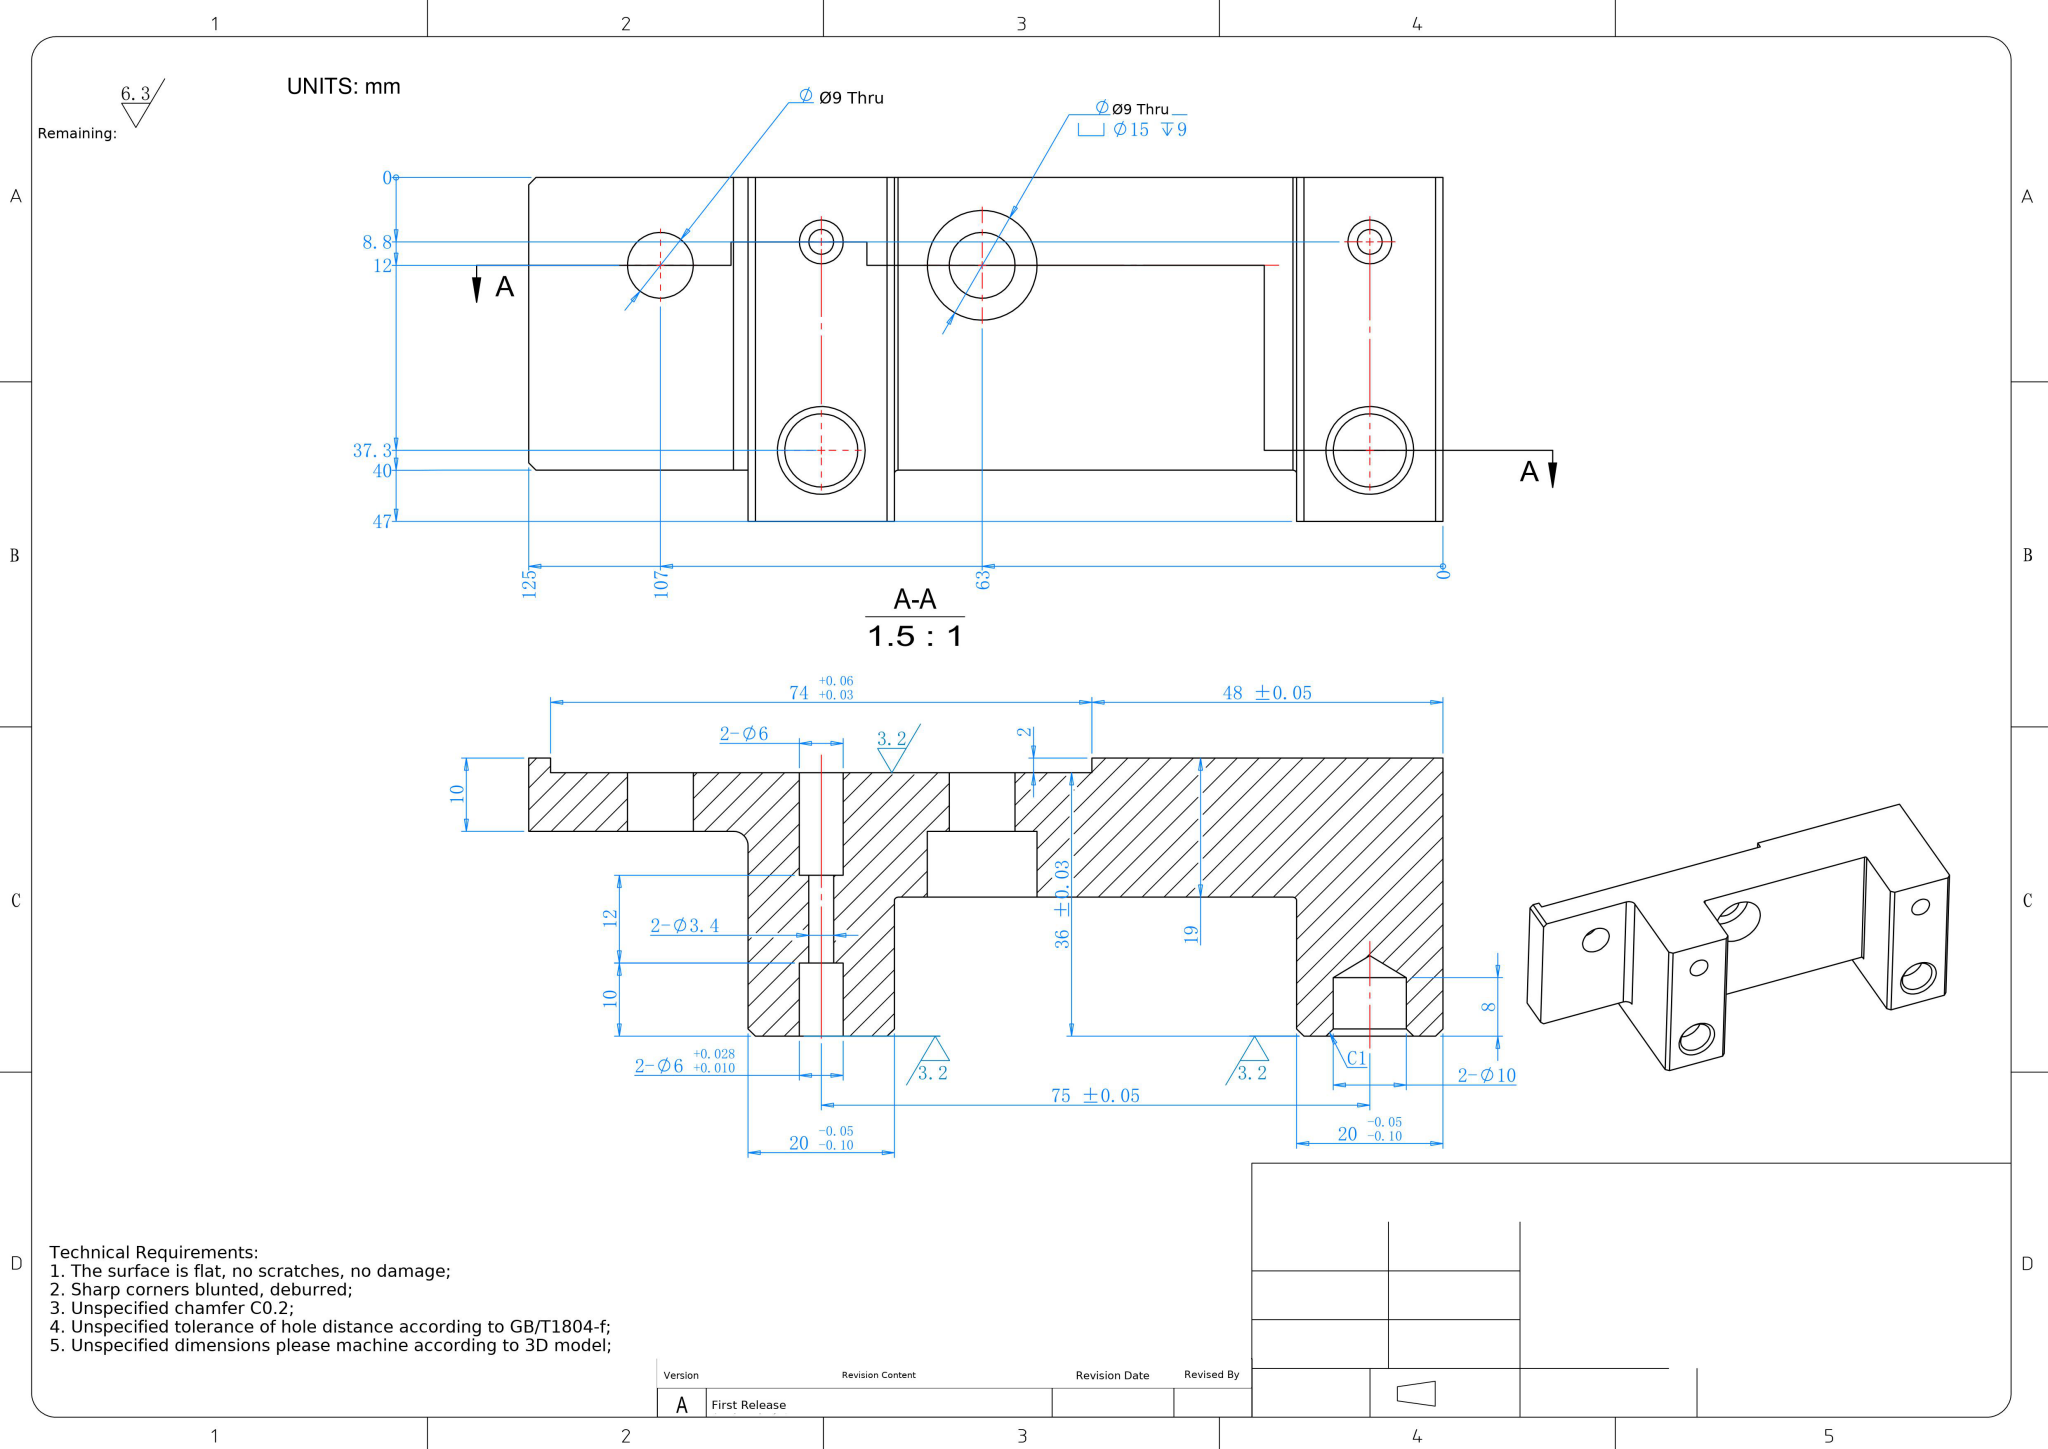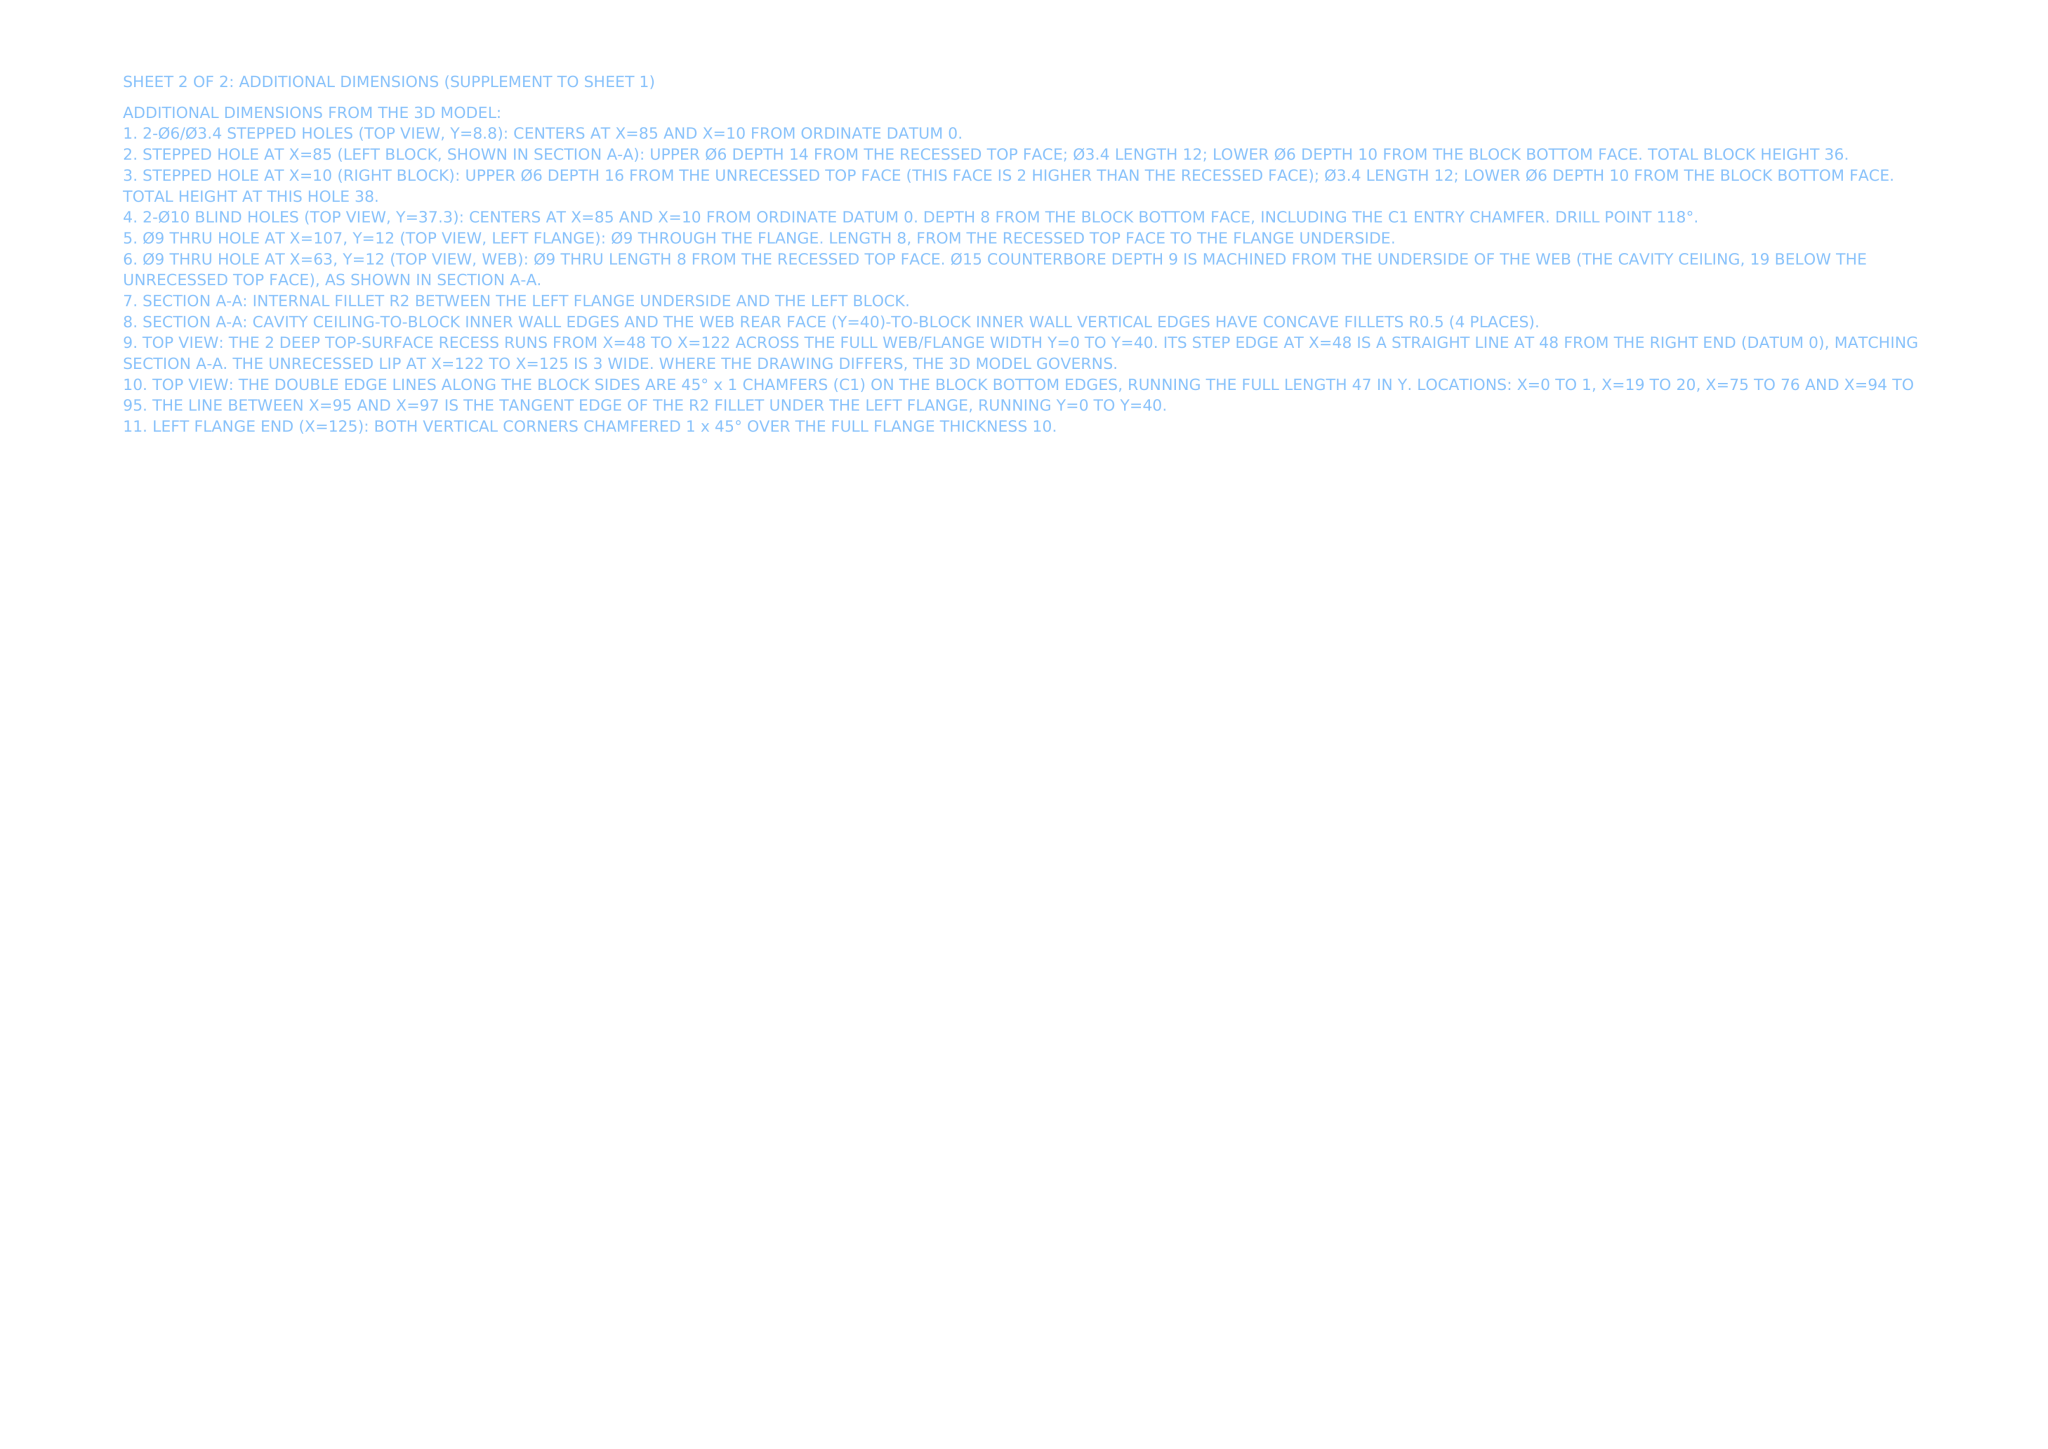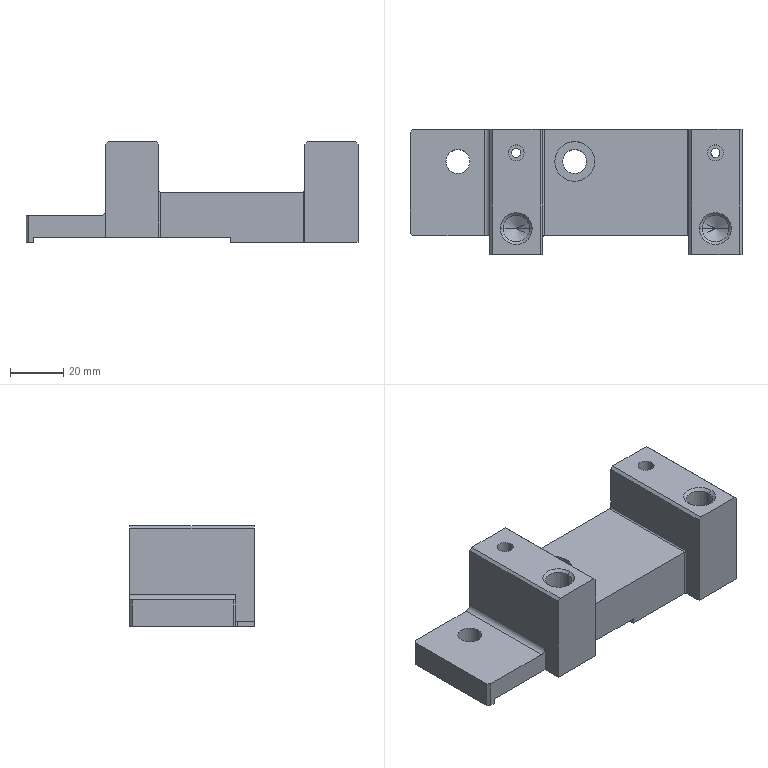Part | NX | mm | 1 solid | 65 faces | box 125 x 47 x 38 mm | volume 113289 mm3 | plane 30 | cylinder 27 | cone 8 | commonest cylinder face diameters 6 x8 9 x4 10 x4 3.4 x4 1 x4 15 x2 4 x1